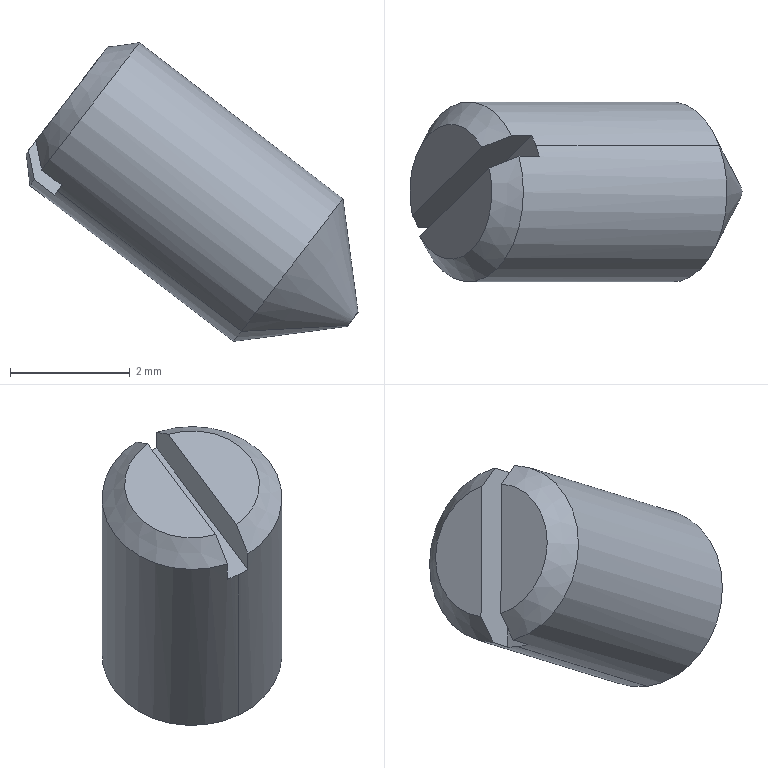Component | SolidWorks | 8-1 | 1 solid | 12 faces | box 5.54 x 3 x 4.98 mm | volume 35 mm3 | plane 6 | cone 4 | cylinder 2 | commonest cylinder face diameters 3 x2
STEP:
#1=COLOUR_RGB('',0.7922,0.8196,0.9333);
#2=FILL_AREA_STYLE_COLOUR('',#1);
#3=FILL_AREA_STYLE('',(#2));
#4=SURFACE_STYLE_FILL_AREA(#3);
#5=SURFACE_SIDE_STYLE('',(#4));
#6=SURFACE_STYLE_USAGE(.BOTH.,#5);
#7=PRESENTATION_STYLE_ASSIGNMENT((#6));
#8=CARTESIAN_POINT('',(-0.6051,-12.852,0.5275));
#9=VERTEX_POINT('',#8);
#10=CARTESIAN_POINT('',(-0.6668,-12.912,0.447));
#11=VERTEX_POINT('',#10);
#12=CARTESIAN_POINT('',(-0.636,-12.882,0.4872));
#13=DIRECTION('',(-0.7938,-0.,0.6082));
#14=DIRECTION('',(0.5225,0.5118,0.682));
#15=AXIS2_PLACEMENT_3D('',#12,#13,#14);
#16=CIRCLE('',#15,0.05906);
#17=EDGE_CURVE('',#9,#11,#16,.T.);
#18=ORIENTED_EDGE('',*,*,#17,.T.);
#19=CARTESIAN_POINT('',(-0.7872,-12.912,0.5391));
#20=VERTEX_POINT('',#19);
#21=CARTESIAN_POINT('',(-1.274,-12.912,0.912));
#22=DIRECTION('',(-0.7938,-0.,0.6082));
#23=VECTOR('',#22,39.37);
#24=LINE('',#21,#23);
#25=EDGE_CURVE('',#11,#20,#24,.T.);
#26=ORIENTED_EDGE('',*,*,#25,.T.);
#27=CARTESIAN_POINT('',(-0.7893,-12.905,0.5363));
#28=VERTEX_POINT('',#27);
#29=CARTESIAN_POINT('',(-0.7563,-12.882,0.5794));
#30=DIRECTION('',(0.7938,0.,-0.6082));
#31=DIRECTION('',(-0.5225,-0.5118,-0.682));
#32=AXIS2_PLACEMENT_3D('',#29,#30,#31);
#33=CIRCLE('',#32,0.05906);
#34=EDGE_CURVE('',#20,#28,#33,.T.);
#35=ORIENTED_EDGE('',*,*,#34,.T.);
#36=CARTESIAN_POINT('',(-0.8026,-12.905,0.5465));
#37=VERTEX_POINT('',#36);
#38=CARTESIAN_POINT('',(-1.276,-12.905,0.9092));
#39=DIRECTION('',(-0.7938,-0.,0.6082));
#40=VECTOR('',#39,39.37);
#41=LINE('',#38,#40);
#42=EDGE_CURVE('',#28,#37,#41,.T.);
#43=ORIENTED_EDGE('',*,*,#42,.T.);
#44=CARTESIAN_POINT('',(-0.7415,-12.845,0.6263));
#45=VERTEX_POINT('',#44);
#46=CARTESIAN_POINT('',(-0.7696,-12.882,0.5896));
#47=DIRECTION('',(-0.7938,-0.,0.6082));
#48=DIRECTION('',(0.5225,0.5118,0.682));
#49=AXIS2_PLACEMENT_3D('',#46,#47,#48);
#50=CIRCLE('',#49,0.05906);
#51=EDGE_CURVE('',#45,#37,#50,.T.);
#52=ORIENTED_EDGE('',*,*,#51,.F.);
#53=CARTESIAN_POINT('',(-0.7282,-12.845,0.6161));
#54=VERTEX_POINT('',#53);
#55=CARTESIAN_POINT('',(-1.215,-12.845,0.989));
#56=DIRECTION('',(0.7938,0.,-0.6082));
#57=VECTOR('',#56,39.37);
#58=LINE('',#55,#57);
#59=EDGE_CURVE('',#45,#54,#58,.T.);
#60=ORIENTED_EDGE('',*,*,#59,.T.);
#61=CARTESIAN_POINT('',(-0.7255,-12.852,0.6197));
#62=VERTEX_POINT('',#61);
#63=CARTESIAN_POINT('',(-0.7563,-12.882,0.5794));
#64=DIRECTION('',(0.7938,0.,-0.6082));
#65=DIRECTION('',(-0.5225,-0.5118,-0.682));
#66=AXIS2_PLACEMENT_3D('',#63,#64,#65);
#67=CIRCLE('',#66,0.05906);
#68=EDGE_CURVE('',#54,#62,#67,.T.);
#69=ORIENTED_EDGE('',*,*,#68,.T.);
#70=CARTESIAN_POINT('',(-1.212,-12.852,0.9926));
#71=DIRECTION('',(-0.7938,-0.,0.6082));
#72=VECTOR('',#71,39.37);
#73=LINE('',#70,#72);
#74=EDGE_CURVE('',#9,#62,#73,.T.);
#75=ORIENTED_EDGE('',*,*,#74,.F.);
#76=EDGE_LOOP('',(#18,#26,#35,#43,#52,#60,#69,#75));
#77=FACE_OUTER_BOUND('',#76,.T.);
#78=CARTESIAN_POINT('',(-1.243,-12.882,0.9523));
#79=DIRECTION('',(-0.7938,-0.,0.6082));
#80=DIRECTION('',(0.5225,0.5118,0.682));
#81=AXIS2_PLACEMENT_3D('',#78,#79,#80);
#82=CYLINDRICAL_SURFACE('',#81,0.05906);
#83=ADVANCED_FACE('',(#77),#82,.T.);
#84=CARTESIAN_POINT('',(-0.5907,-12.879,0.4589));
#85=VERTEX_POINT('',#84);
#86=CARTESIAN_POINT('',(-0.5969,-12.885,0.4509));
#87=VERTEX_POINT('',#86);
#88=CARTESIAN_POINT('',(-0.5938,-12.882,0.4549));
#89=DIRECTION('',(-0.7938,-0.,0.6082));
#90=DIRECTION('',(0.5225,0.5118,0.682));
#91=AXIS2_PLACEMENT_3D('',#88,#89,#90);
#92=CIRCLE('',#91,0.005906);
#93=EDGE_CURVE('',#85,#87,#92,.T.);
#94=ORIENTED_EDGE('',*,*,#93,.T.);
#95=CARTESIAN_POINT('',(-0.5969,-12.885,0.4509));
#96=DIRECTION('',(-0.9307,-0.3619,-0.05219));
#97=VECTOR('',#96,39.37);
#98=LINE('',#95,#97);
#99=EDGE_CURVE('',#87,#11,#98,.T.);
#100=ORIENTED_EDGE('',*,*,#99,.T.);
#101=ORIENTED_EDGE('',*,*,#17,.F.);
#102=CARTESIAN_POINT('',(-0.5907,-12.879,0.4589));
#103=DIRECTION('',(-0.1919,0.3619,0.9122));
#104=VECTOR('',#103,39.37);
#105=LINE('',#102,#104);
#106=EDGE_CURVE('',#85,#9,#105,.T.);
#107=ORIENTED_EDGE('',*,*,#106,.F.);
#108=EDGE_LOOP('',(#94,#100,#101,#107));
#109=FACE_OUTER_BOUND('',#108,.T.);
#110=CARTESIAN_POINT('',(-0.5938,-12.882,0.4549));
#111=DIRECTION('',(-0.7938,-0.,0.6082));
#112=DIRECTION('',(0.5225,0.5118,0.682));
#113=AXIS2_PLACEMENT_3D('',#110,#111,#112);
#114=CONICAL_SURFACE('',#113,0.005906,0.7854);
#115=ADVANCED_FACE('',(#109),#114,.T.);
#116=CARTESIAN_POINT('',(-0.761,-12.853,0.6251));
#117=VERTEX_POINT('',#116);
#118=CARTESIAN_POINT('',(-0.8065,-12.897,0.5657));
#119=VERTEX_POINT('',#118);
#120=CARTESIAN_POINT('',(-0.7813,-12.882,0.5986));
#121=DIRECTION('',(-0.7938,-0.,0.6082));
#122=DIRECTION('',(0.5225,0.5118,0.682));
#123=AXIS2_PLACEMENT_3D('',#120,#121,#122);
#124=CIRCLE('',#123,0.04429);
#125=EDGE_CURVE('',#117,#119,#124,.T.);
#126=ORIENTED_EDGE('',*,*,#125,.T.);
#127=CARTESIAN_POINT('',(-0.8146,-12.905,0.5551));
#128=DIRECTION('',(0.5225,0.5118,0.682));
#129=VECTOR('',#128,39.37);
#130=LINE('',#127,#129);
#131=EDGE_CURVE('',#119,#117,#130,.T.);
#132=ORIENTED_EDGE('',*,*,#131,.T.);
#133=EDGE_LOOP('',(#126,#132));
#134=FACE_OUTER_BOUND('',#133,.T.);
#135=CARTESIAN_POINT('',(-0.7951,-12.844,0.5806));
#136=DIRECTION('',(0.7938,0.,-0.6082));
#137=DIRECTION('',(-0.5225,-0.5118,-0.682));
#138=AXIS2_PLACEMENT_3D('',#135,#136,#137);
#139=PLANE('',#138);
#140=ADVANCED_FACE('',(#134),#139,.F.);
#141=ORIENTED_EDGE('',*,*,#51,.T.);
#142=CARTESIAN_POINT('',(-0.8026,-12.905,0.5465));
#143=CARTESIAN_POINT('',(-0.8039,-12.903,0.5529));
#144=CARTESIAN_POINT('',(-0.8052,-12.9,0.5593));
#145=CARTESIAN_POINT('',(-0.8065,-12.897,0.5657));
#146=B_SPLINE_CURVE_WITH_KNOTS('',3,(#142,#143,#144,#145),.UNSPECIFIED.,.F.,.F.,(4,4),(0.002571,0.003104),.UNSPECIFIED.);
#147=EDGE_CURVE('',#37,#119,#146,.T.);
#148=ORIENTED_EDGE('',*,*,#147,.T.);
#149=ORIENTED_EDGE('',*,*,#125,.F.);
#150=CARTESIAN_POINT('',(-0.761,-12.853,0.6251));
#151=CARTESIAN_POINT('',(-0.7545,-12.85,0.6255));
#152=CARTESIAN_POINT('',(-0.748,-12.848,0.6259));
#153=CARTESIAN_POINT('',(-0.7415,-12.845,0.6263));
#154=B_SPLINE_CURVE_WITH_KNOTS('',3,(#150,#151,#152,#153),.UNSPECIFIED.,.F.,.F.,(4,4),(0.006025,0.00656),.UNSPECIFIED.);
#155=EDGE_CURVE('',#117,#45,#154,.T.);
#156=ORIENTED_EDGE('',*,*,#155,.T.);
#157=EDGE_LOOP('',(#141,#148,#149,#156));
#158=FACE_OUTER_BOUND('',#157,.T.);
#159=CARTESIAN_POINT('',(-0.7696,-12.882,0.5896));
#160=DIRECTION('',(0.7938,0.,-0.6082));
#161=DIRECTION('',(-0.5225,-0.5118,-0.682));
#162=AXIS2_PLACEMENT_3D('',#159,#160,#161);
#163=CONICAL_SURFACE('',#162,0.05906,0.7854);
#164=ADVANCED_FACE('',(#158),#163,.T.);
#165=CARTESIAN_POINT('',(-0.8016,-12.911,0.5721));
#166=VERTEX_POINT('',#165);
#167=CARTESIAN_POINT('',(-0.7561,-12.866,0.6315));
#168=VERTEX_POINT('',#167);
#169=CARTESIAN_POINT('',(-0.7813,-12.882,0.5986));
#170=DIRECTION('',(-0.7938,-0.,0.6082));
#171=DIRECTION('',(0.5225,0.5118,0.682));
#172=AXIS2_PLACEMENT_3D('',#169,#170,#171);
#173=CIRCLE('',#172,0.04429);
#174=EDGE_CURVE('',#166,#168,#173,.T.);
#175=ORIENTED_EDGE('',*,*,#174,.T.);
#176=CARTESIAN_POINT('',(-0.8097,-12.919,0.5615));
#177=DIRECTION('',(0.5225,0.5118,0.682));
#178=VECTOR('',#177,39.37);
#179=LINE('',#176,#178);
#180=EDGE_CURVE('',#166,#168,#179,.T.);
#181=ORIENTED_EDGE('',*,*,#180,.F.);
#182=EDGE_LOOP('',(#175,#181));
#183=FACE_OUTER_BOUND('',#182,.T.);
#184=CARTESIAN_POINT('',(-0.7951,-12.844,0.5806));
#185=DIRECTION('',(0.7938,0.,-0.6082));
#186=DIRECTION('',(-0.5225,-0.5118,-0.682));
#187=AXIS2_PLACEMENT_3D('',#184,#185,#186);
#188=PLANE('',#187);
#189=ADVANCED_FACE('',(#183),#188,.F.);
#190=ORIENTED_EDGE('',*,*,#93,.F.);
#191=CARTESIAN_POINT('',(-0.5938,-12.882,0.4549));
#192=DIRECTION('',(-0.7938,-0.,0.6082));
#193=DIRECTION('',(0.5225,0.5118,0.682));
#194=AXIS2_PLACEMENT_3D('',#191,#192,#193);
#195=CIRCLE('',#194,0.005906);
#196=EDGE_CURVE('',#87,#85,#195,.T.);
#197=ORIENTED_EDGE('',*,*,#196,.F.);
#198=EDGE_LOOP('',(#190,#197));
#199=FACE_OUTER_BOUND('',#198,.T.);
#200=CARTESIAN_POINT('',(-0.5938,-12.882,0.4549));
#201=DIRECTION('',(-0.7938,-0.,0.6082));
#202=DIRECTION('',(0.5225,0.5118,0.682));
#203=AXIS2_PLACEMENT_3D('',#200,#201,#202);
#204=PLANE('',#203);
#205=ADVANCED_FACE('',(#199),#204,.F.);
#206=ORIENTED_EDGE('',*,*,#99,.F.);
#207=ORIENTED_EDGE('',*,*,#196,.T.);
#208=ORIENTED_EDGE('',*,*,#106,.T.);
#209=CARTESIAN_POINT('',(-0.636,-12.882,0.4872));
#210=DIRECTION('',(-0.7938,-0.,0.6082));
#211=DIRECTION('',(0.5225,0.5118,0.682));
#212=AXIS2_PLACEMENT_3D('',#209,#210,#211);
#213=CIRCLE('',#212,0.05906);
#214=EDGE_CURVE('',#11,#9,#213,.T.);
#215=ORIENTED_EDGE('',*,*,#214,.F.);
#216=EDGE_LOOP('',(#206,#207,#208,#215));
#217=FACE_OUTER_BOUND('',#216,.T.);
#218=CARTESIAN_POINT('',(-0.5938,-12.882,0.4549));
#219=DIRECTION('',(-0.7938,-0.,0.6082));
#220=DIRECTION('',(0.5225,0.5118,0.682));
#221=AXIS2_PLACEMENT_3D('',#218,#219,#220);
#222=CONICAL_SURFACE('',#221,0.005906,0.7854);
#223=ADVANCED_FACE('',(#217),#222,.T.);
#224=ORIENTED_EDGE('',*,*,#25,.F.);
#225=ORIENTED_EDGE('',*,*,#214,.T.);
#226=ORIENTED_EDGE('',*,*,#74,.T.);
#227=CARTESIAN_POINT('',(-0.7233,-12.859,0.6225));
#228=VERTEX_POINT('',#227);
#229=CARTESIAN_POINT('',(-0.7563,-12.882,0.5794));
#230=DIRECTION('',(0.7938,0.,-0.6082));
#231=DIRECTION('',(-0.5225,-0.5118,-0.682));
#232=AXIS2_PLACEMENT_3D('',#229,#230,#231);
#233=CIRCLE('',#232,0.05906);
#234=EDGE_CURVE('',#62,#228,#233,.T.);
#235=ORIENTED_EDGE('',*,*,#234,.T.);
#236=CARTESIAN_POINT('',(-0.7366,-12.859,0.6327));
#237=VERTEX_POINT('',#236);
#238=CARTESIAN_POINT('',(-1.21,-12.859,0.9954));
#239=DIRECTION('',(-0.7938,-0.,0.6082));
#240=VECTOR('',#239,39.37);
#241=LINE('',#238,#240);
#242=EDGE_CURVE('',#228,#237,#241,.T.);
#243=ORIENTED_EDGE('',*,*,#242,.T.);
#244=CARTESIAN_POINT('',(-0.7977,-12.919,0.5529));
#245=VERTEX_POINT('',#244);
#246=CARTESIAN_POINT('',(-0.7696,-12.882,0.5896));
#247=DIRECTION('',(-0.7938,-0.,0.6082));
#248=DIRECTION('',(0.5225,0.5118,0.682));
#249=AXIS2_PLACEMENT_3D('',#246,#247,#248);
#250=CIRCLE('',#249,0.05906);
#251=EDGE_CURVE('',#245,#237,#250,.T.);
#252=ORIENTED_EDGE('',*,*,#251,.F.);
#253=CARTESIAN_POINT('',(-0.7844,-12.919,0.5427));
#254=VERTEX_POINT('',#253);
#255=CARTESIAN_POINT('',(-1.271,-12.919,0.9156));
#256=DIRECTION('',(0.7938,0.,-0.6082));
#257=VECTOR('',#256,39.37);
#258=LINE('',#255,#257);
#259=EDGE_CURVE('',#245,#254,#258,.T.);
#260=ORIENTED_EDGE('',*,*,#259,.T.);
#261=CARTESIAN_POINT('',(-0.7563,-12.882,0.5794));
#262=DIRECTION('',(0.7938,0.,-0.6082));
#263=DIRECTION('',(-0.5225,-0.5118,-0.682));
#264=AXIS2_PLACEMENT_3D('',#261,#262,#263);
#265=CIRCLE('',#264,0.05906);
#266=EDGE_CURVE('',#254,#20,#265,.T.);
#267=ORIENTED_EDGE('',*,*,#266,.T.);
#268=EDGE_LOOP('',(#224,#225,#226,#235,#243,#252,#260,#267));
#269=FACE_OUTER_BOUND('',#268,.T.);
#270=CARTESIAN_POINT('',(-1.243,-12.882,0.9523));
#271=DIRECTION('',(-0.7938,-0.,0.6082));
#272=DIRECTION('',(0.5225,0.5118,0.682));
#273=AXIS2_PLACEMENT_3D('',#270,#271,#272);
#274=CYLINDRICAL_SURFACE('',#273,0.05906);
#275=ADVANCED_FACE('',(#269),#274,.T.);
#276=ORIENTED_EDGE('',*,*,#251,.T.);
#277=CARTESIAN_POINT('',(-0.7366,-12.859,0.6327));
#278=CARTESIAN_POINT('',(-0.7431,-12.861,0.6323));
#279=CARTESIAN_POINT('',(-0.7496,-12.864,0.6319));
#280=CARTESIAN_POINT('',(-0.7561,-12.866,0.6315));
#281=B_SPLINE_CURVE_WITH_KNOTS('',3,(#277,#278,#279,#280),.UNSPECIFIED.,.F.,.F.,(4,4),(0.002571,0.003104),.UNSPECIFIED.);
#282=EDGE_CURVE('',#237,#168,#281,.T.);
#283=ORIENTED_EDGE('',*,*,#282,.T.);
#284=ORIENTED_EDGE('',*,*,#174,.F.);
#285=CARTESIAN_POINT('',(-0.8016,-12.911,0.5721));
#286=CARTESIAN_POINT('',(-0.8003,-12.914,0.5657));
#287=CARTESIAN_POINT('',(-0.799,-12.916,0.5593));
#288=CARTESIAN_POINT('',(-0.7977,-12.919,0.5529));
#289=B_SPLINE_CURVE_WITH_KNOTS('',3,(#285,#286,#287,#288),.UNSPECIFIED.,.F.,.F.,(4,4),(0.006025,0.00656),.UNSPECIFIED.);
#290=EDGE_CURVE('',#166,#245,#289,.T.);
#291=ORIENTED_EDGE('',*,*,#290,.T.);
#292=EDGE_LOOP('',(#276,#283,#284,#291));
#293=FACE_OUTER_BOUND('',#292,.T.);
#294=CARTESIAN_POINT('',(-0.7696,-12.882,0.5896));
#295=DIRECTION('',(0.7938,0.,-0.6082));
#296=DIRECTION('',(-0.5225,-0.5118,-0.682));
#297=AXIS2_PLACEMENT_3D('',#294,#295,#296);
#298=CONICAL_SURFACE('',#297,0.05906,0.7854);
#299=ADVANCED_FACE('',(#293),#298,.T.);
#300=CARTESIAN_POINT('',(-0.7896,-12.905,0.5359));
#301=DIRECTION('',(0.5225,0.5118,0.682));
#302=VECTOR('',#301,39.37);
#303=LINE('',#300,#302);
#304=EDGE_CURVE('',#28,#54,#303,.T.);
#305=ORIENTED_EDGE('',*,*,#304,.F.);
#306=ORIENTED_EDGE('',*,*,#34,.F.);
#307=ORIENTED_EDGE('',*,*,#266,.F.);
#308=CARTESIAN_POINT('',(-0.7847,-12.919,0.5423));
#309=DIRECTION('',(0.5225,0.5118,0.682));
#310=VECTOR('',#309,39.37);
#311=LINE('',#308,#310);
#312=EDGE_CURVE('',#254,#228,#311,.T.);
#313=ORIENTED_EDGE('',*,*,#312,.T.);
#314=ORIENTED_EDGE('',*,*,#234,.F.);
#315=ORIENTED_EDGE('',*,*,#68,.F.);
#316=EDGE_LOOP('',(#305,#306,#307,#313,#314,#315));
#317=FACE_OUTER_BOUND('',#316,.T.);
#318=CARTESIAN_POINT('',(-0.7896,-12.905,0.5359));
#319=DIRECTION('',(0.7938,0.,-0.6082));
#320=DIRECTION('',(-0.5225,-0.5118,-0.682));
#321=AXIS2_PLACEMENT_3D('',#318,#319,#320);
#322=PLANE('',#321);
#323=ADVANCED_FACE('',(#317),#322,.F.);
#324=ORIENTED_EDGE('',*,*,#304,.T.);
#325=ORIENTED_EDGE('',*,*,#59,.F.);
#326=ORIENTED_EDGE('',*,*,#155,.F.);
#327=ORIENTED_EDGE('',*,*,#131,.F.);
#328=ORIENTED_EDGE('',*,*,#147,.F.);
#329=ORIENTED_EDGE('',*,*,#42,.F.);
#330=EDGE_LOOP('',(#324,#325,#326,#327,#328,#329));
#331=FACE_OUTER_BOUND('',#330,.T.);
#332=CARTESIAN_POINT('',(-0.8146,-12.905,0.5551));
#333=DIRECTION('',(-0.3113,0.8591,-0.4063));
#334=DIRECTION('',(0.5225,0.5118,0.682));
#335=AXIS2_PLACEMENT_3D('',#332,#333,#334);
#336=PLANE('',#335);
#337=ADVANCED_FACE('',(#331),#336,.F.);
#338=ORIENTED_EDGE('',*,*,#312,.F.);
#339=ORIENTED_EDGE('',*,*,#259,.F.);
#340=ORIENTED_EDGE('',*,*,#290,.F.);
#341=ORIENTED_EDGE('',*,*,#180,.T.);
#342=ORIENTED_EDGE('',*,*,#282,.F.);
#343=ORIENTED_EDGE('',*,*,#242,.F.);
#344=EDGE_LOOP('',(#338,#339,#340,#341,#342,#343));
#345=FACE_OUTER_BOUND('',#344,.T.);
#346=CARTESIAN_POINT('',(-0.8097,-12.919,0.5615));
#347=DIRECTION('',(0.3113,-0.8591,0.4063));
#348=DIRECTION('',(-0.5225,-0.5118,-0.682));
#349=AXIS2_PLACEMENT_3D('',#346,#347,#348);
#350=PLANE('',#349);
#351=ADVANCED_FACE('',(#345),#350,.F.);
#352=CLOSED_SHELL('',(#83,#115,#140,#164,#189,#205,#223,#275,#299,#323,#337,#351));
#353=MANIFOLD_SOLID_BREP('',#352);
#354=STYLED_ITEM('',(#7),#353);
#355=(LENGTH_UNIT()NAMED_UNIT(*)SI_UNIT($,.METRE.));
#356=LENGTH_MEASURE_WITH_UNIT(LENGTH_MEASURE(0.0254),#355);
#357=DIMENSIONAL_EXPONENTS(1.,0.,0.,0.,0.,0.,0.);
#358=(CONVERSION_BASED_UNIT('',#356)LENGTH_UNIT()NAMED_UNIT(#357));
#359=UNCERTAINTY_MEASURE_WITH_UNIT(LENGTH_MEASURE(0.00001),#358,'','');
#360=(NAMED_UNIT(*)PLANE_ANGLE_UNIT()SI_UNIT($,.RADIAN.));
#361=(NAMED_UNIT(*)SI_UNIT($,.STERADIAN.)SOLID_ANGLE_UNIT());
#362=(GEOMETRIC_REPRESENTATION_CONTEXT(3)GLOBAL_UNCERTAINTY_ASSIGNED_CONTEXT((#359))GLOBAL_UNIT_ASSIGNED_CONTEXT((#358,#360,#361))REPRESENTATION_CONTEXT('',''));
#363=MECHANICAL_DESIGN_GEOMETRIC_PRESENTATION_REPRESENTATION('',(#354),#362);
#364=PRESENTATION_LAYER_ASSIGNMENT('','',(#354));
#365=CARTESIAN_POINT('',(0.,0.,0.));
#366=DIRECTION('',(0.,0.,1.));
#367=DIRECTION('',(1.,0.,0.));
#368=AXIS2_PLACEMENT_3D('',#365,#366,#367);
#369=(LENGTH_UNIT()NAMED_UNIT(*)SI_UNIT($,.METRE.));
#370=LENGTH_MEASURE_WITH_UNIT(LENGTH_MEASURE(0.0254),#369);
#371=DIMENSIONAL_EXPONENTS(1.,0.,0.,0.,0.,0.,0.);
#372=(CONVERSION_BASED_UNIT('',#370)LENGTH_UNIT()NAMED_UNIT(#371));
#373=UNCERTAINTY_MEASURE_WITH_UNIT(LENGTH_MEASURE(0.00001),#372,'','');
#374=(NAMED_UNIT(*)PLANE_ANGLE_UNIT()SI_UNIT($,.RADIAN.));
#375=(NAMED_UNIT(*)SI_UNIT($,.STERADIAN.)SOLID_ANGLE_UNIT());
#376=(GEOMETRIC_REPRESENTATION_CONTEXT(3)GLOBAL_UNCERTAINTY_ASSIGNED_CONTEXT((#373))GLOBAL_UNIT_ASSIGNED_CONTEXT((#372,#374,#375))REPRESENTATION_CONTEXT('',''));
#377=ADVANCED_BREP_SHAPE_REPRESENTATION('',(#353,#368),#376);